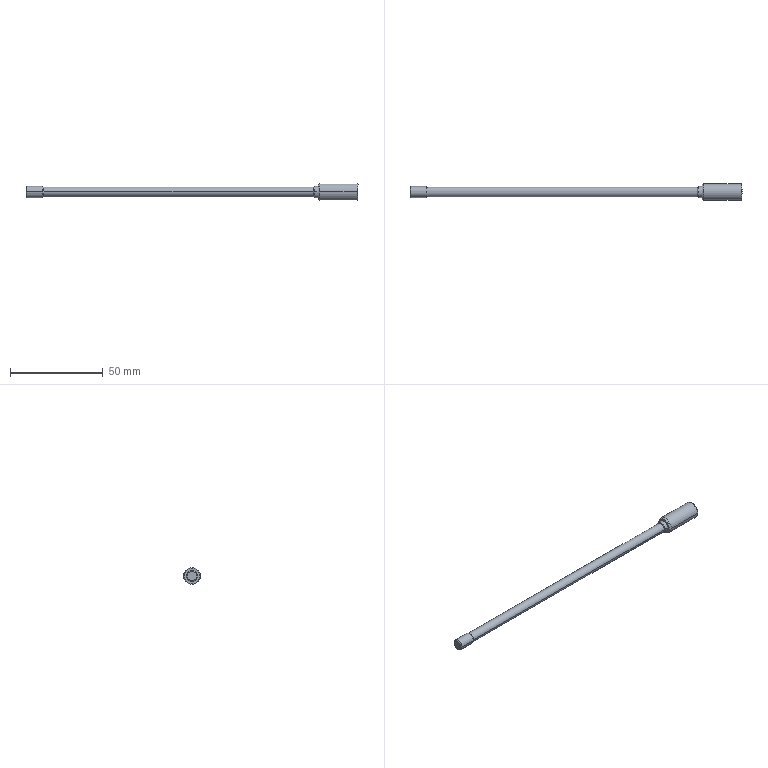Component | SolidWorks | HZ022-SC32x100S-1_HZ022-SC32x100S (5)-1 | 1 solid | 38 faces | box 178.5 x 9 x 9 mm | volume 4474 mm3 | plane 16 | cylinder 10 | cone 10 | spline 2 | commonest cylinder face diameters 6 x4 5.22 x2 9 x2 4.917 x2 | material AL6061
STEP:
#1=COLOUR_RGB('',0.7922,0.8196,0.9333);
#2=FILL_AREA_STYLE_COLOUR('',#1);
#3=FILL_AREA_STYLE('',(#2));
#4=SURFACE_STYLE_FILL_AREA(#3);
#5=SURFACE_SIDE_STYLE('',(#4));
#6=SURFACE_STYLE_USAGE(.BOTH.,#5);
#7=PRESENTATION_STYLE_ASSIGNMENT((#6));
#8=CARTESIAN_POINT('',(-3.546,5.478,37.146));
#9=VERTEX_POINT('',#8);
#10=CARTESIAN_POINT('',(-3.546,5.793,37.146));
#11=VERTEX_POINT('',#10);
#12=CARTESIAN_POINT('',(-3.546,5.478,37.146));
#13=CARTESIAN_POINT('',(-3.546,5.478,37.461));
#14=CARTESIAN_POINT('',(-3.546,5.793,37.461));
#15=CARTESIAN_POINT('',(-3.546,5.793,37.146));
#16=(BOUNDED_CURVE()B_SPLINE_CURVE(3,(#12,#13,#14,#15),.UNSPECIFIED.,.F.,.F.)B_SPLINE_CURVE_WITH_KNOTS((4,4),(0.,1.),.UNSPECIFIED.)CURVE()GEOMETRIC_REPRESENTATION_ITEM()RATIONAL_B_SPLINE_CURVE((1.,0.3333,0.3333,1.))REPRESENTATION_ITEM(''));
#17=EDGE_CURVE('',#9,#11,#16,.T.);
#18=ORIENTED_EDGE('',*,*,#17,.T.);
#19=CARTESIAN_POINT('',(-3.565,5.813,37.146));
#20=VERTEX_POINT('',#19);
#21=CARTESIAN_POINT('',(-3.565,5.793,37.146));
#22=DIRECTION('',(0.,0.,1.));
#23=DIRECTION('',(0.,1.,0.));
#24=AXIS2_PLACEMENT_3D('',#21,#22,#23);
#25=CIRCLE('',#24,0.01969);
#26=EDGE_CURVE('',#11,#20,#25,.T.);
#27=ORIENTED_EDGE('',*,*,#26,.T.);
#28=CARTESIAN_POINT('',(-3.565,5.459,37.146));
#29=VERTEX_POINT('',#28);
#30=CARTESIAN_POINT('',(-3.565,5.636,37.146));
#31=DIRECTION('',(-1.,-0.,0.));
#32=DIRECTION('',(0.,1.,0.));
#33=AXIS2_PLACEMENT_3D('',#30,#31,#32);
#34=CIRCLE('',#33,0.1772);
#35=EDGE_CURVE('',#29,#20,#34,.T.);
#36=ORIENTED_EDGE('',*,*,#35,.F.);
#37=CARTESIAN_POINT('',(-3.565,5.478,37.146));
#38=DIRECTION('',(-0.,0.,-1.));
#39=DIRECTION('',(0.,-1.,0.));
#40=AXIS2_PLACEMENT_3D('',#37,#38,#39);
#41=CIRCLE('',#40,0.01969);
#42=EDGE_CURVE('',#9,#29,#41,.T.);
#43=ORIENTED_EDGE('',*,*,#42,.F.);
#44=EDGE_LOOP('',(#18,#27,#36,#43));
#45=FACE_OUTER_BOUND('',#44,.T.);
#46=CARTESIAN_POINT('',(-3.546,5.793,37.146));
#47=CARTESIAN_POINT('',(-3.546,5.793,37.461));
#48=CARTESIAN_POINT('',(-3.546,5.478,37.461));
#49=CARTESIAN_POINT('',(-3.546,5.478,37.146));
#50=CARTESIAN_POINT('',(-3.546,5.805,37.146));
#51=CARTESIAN_POINT('',(-3.546,5.805,37.484));
#52=CARTESIAN_POINT('',(-3.546,5.467,37.484));
#53=CARTESIAN_POINT('',(-3.546,5.467,37.146));
#54=CARTESIAN_POINT('',(-3.554,5.813,37.146));
#55=CARTESIAN_POINT('',(-3.554,5.813,37.5));
#56=CARTESIAN_POINT('',(-3.554,5.459,37.5));
#57=CARTESIAN_POINT('',(-3.554,5.459,37.146));
#58=CARTESIAN_POINT('',(-3.565,5.813,37.146));
#59=CARTESIAN_POINT('',(-3.565,5.813,37.5));
#60=CARTESIAN_POINT('',(-3.565,5.459,37.5));
#61=CARTESIAN_POINT('',(-3.565,5.459,37.146));
#62=(BOUNDED_SURFACE()B_SPLINE_SURFACE(3,3,((#46,#47,#48,#49),(#50,#51,#52,#53),(#54,#55,#56,#57),(#58,#59,#60,#61)),.UNSPECIFIED.,.F.,.F.,.T.)B_SPLINE_SURFACE_WITH_KNOTS((4,4),(4,4),(0.,1.),(0.,1.),.UNSPECIFIED.)GEOMETRIC_REPRESENTATION_ITEM()RATIONAL_B_SPLINE_SURFACE(((1.,0.3333,0.3333,1.),(0.8047,0.2682,0.2682,0.8047),(0.8047,0.2682,0.2682,0.8047),(1.,0.3333,0.3333,1.)))REPRESENTATION_ITEM('')SURFACE());
#63=ADVANCED_FACE('',(#45),#62,.T.);
#64=CARTESIAN_POINT('',(-4.49,5.739,37.146));
#65=VERTEX_POINT('',#64);
#66=CARTESIAN_POINT('',(-4.49,5.533,37.146));
#67=VERTEX_POINT('',#66);
#68=CARTESIAN_POINT('',(-4.49,5.636,37.146));
#69=DIRECTION('',(-1.,-0.,0.));
#70=DIRECTION('',(0.,1.,0.));
#71=AXIS2_PLACEMENT_3D('',#68,#69,#70);
#72=CIRCLE('',#71,0.1028);
#73=EDGE_CURVE('',#65,#67,#72,.T.);
#74=ORIENTED_EDGE('',*,*,#73,.T.);
#75=CARTESIAN_POINT('',(-10.199,5.533,37.146));
#76=VERTEX_POINT('',#75);
#77=CARTESIAN_POINT('',(-7.345,5.533,37.146));
#78=DIRECTION('',(-1.,-0.,0.));
#79=VECTOR('',#78,39.37);
#80=LINE('',#77,#79);
#81=EDGE_CURVE('',#67,#76,#80,.T.);
#82=ORIENTED_EDGE('',*,*,#81,.T.);
#83=CARTESIAN_POINT('',(-10.199,5.739,37.146));
#84=VERTEX_POINT('',#83);
#85=CARTESIAN_POINT('',(-10.199,5.636,37.146));
#86=DIRECTION('',(1.,0.,-0.));
#87=DIRECTION('',(0.,1.,0.));
#88=AXIS2_PLACEMENT_3D('',#85,#86,#87);
#89=CIRCLE('',#88,0.1028);
#90=EDGE_CURVE('',#76,#84,#89,.T.);
#91=ORIENTED_EDGE('',*,*,#90,.T.);
#92=CARTESIAN_POINT('',(-7.345,5.739,37.146));
#93=DIRECTION('',(-1.,-0.,0.));
#94=VECTOR('',#93,39.37);
#95=LINE('',#92,#94);
#96=EDGE_CURVE('',#65,#84,#95,.T.);
#97=ORIENTED_EDGE('',*,*,#96,.F.);
#98=EDGE_LOOP('',(#74,#82,#91,#97));
#99=FACE_OUTER_BOUND('',#98,.T.);
#100=CARTESIAN_POINT('',(-7.345,5.636,37.146));
#101=DIRECTION('',(-1.,-0.,0.));
#102=DIRECTION('',(0.,1.,0.));
#103=AXIS2_PLACEMENT_3D('',#100,#101,#102);
#104=CYLINDRICAL_SURFACE('',#103,0.1028);
#105=ADVANCED_FACE('',(#99),#104,.T.);
#106=ORIENTED_EDGE('',*,*,#90,.F.);
#107=CARTESIAN_POINT('',(-10.214,5.518,37.146));
#108=VERTEX_POINT('',#107);
#109=CARTESIAN_POINT('',(-10.214,5.518,37.146));
#110=DIRECTION('',(-0.7071,-0.7071,0.));
#111=VECTOR('',#110,39.37);
#112=LINE('',#109,#111);
#113=EDGE_CURVE('',#76,#108,#112,.T.);
#114=ORIENTED_EDGE('',*,*,#113,.T.);
#115=CARTESIAN_POINT('',(-10.214,5.754,37.146));
#116=VERTEX_POINT('',#115);
#117=CARTESIAN_POINT('',(-10.214,5.636,37.146));
#118=DIRECTION('',(1.,0.,-0.));
#119=DIRECTION('',(-0.,0.,-1.));
#120=AXIS2_PLACEMENT_3D('',#117,#118,#119);
#121=CIRCLE('',#120,0.1181);
#122=EDGE_CURVE('',#108,#116,#121,.T.);
#123=ORIENTED_EDGE('',*,*,#122,.T.);
#124=CARTESIAN_POINT('',(-10.214,5.754,37.146));
#125=DIRECTION('',(-0.7071,0.7071,0.));
#126=VECTOR('',#125,39.37);
#127=LINE('',#124,#126);
#128=EDGE_CURVE('',#84,#116,#127,.T.);
#129=ORIENTED_EDGE('',*,*,#128,.F.);
#130=EDGE_LOOP('',(#106,#114,#123,#129));
#131=FACE_OUTER_BOUND('',#130,.T.);
#132=CARTESIAN_POINT('',(-10.214,5.636,37.146));
#133=DIRECTION('',(-1.,-0.,0.));
#134=DIRECTION('',(0.,1.,0.));
#135=AXIS2_PLACEMENT_3D('',#132,#133,#134);
#136=CONICAL_SURFACE('',#135,0.1181,0.7854);
#137=ADVANCED_FACE('',(#131),#136,.T.);
#138=ORIENTED_EDGE('',*,*,#73,.F.);
#139=CARTESIAN_POINT('',(-4.475,5.754,37.146));
#140=VERTEX_POINT('',#139);
#141=CARTESIAN_POINT('',(-4.475,5.754,37.146));
#142=DIRECTION('',(0.7071,0.7071,-0.));
#143=VECTOR('',#142,39.37);
#144=LINE('',#141,#143);
#145=EDGE_CURVE('',#65,#140,#144,.T.);
#146=ORIENTED_EDGE('',*,*,#145,.T.);
#147=CARTESIAN_POINT('',(-4.475,5.518,37.146));
#148=VERTEX_POINT('',#147);
#149=CARTESIAN_POINT('',(-4.475,5.636,37.146));
#150=DIRECTION('',(-1.,-0.,0.));
#151=DIRECTION('',(-0.,0.,-1.));
#152=AXIS2_PLACEMENT_3D('',#149,#150,#151);
#153=CIRCLE('',#152,0.1181);
#154=EDGE_CURVE('',#140,#148,#153,.T.);
#155=ORIENTED_EDGE('',*,*,#154,.T.);
#156=CARTESIAN_POINT('',(-4.475,5.518,37.146));
#157=DIRECTION('',(0.7071,-0.7071,-0.));
#158=VECTOR('',#157,39.37);
#159=LINE('',#156,#158);
#160=EDGE_CURVE('',#67,#148,#159,.T.);
#161=ORIENTED_EDGE('',*,*,#160,.F.);
#162=EDGE_LOOP('',(#138,#146,#155,#161));
#163=FACE_OUTER_BOUND('',#162,.T.);
#164=CARTESIAN_POINT('',(-4.475,5.636,37.146));
#165=DIRECTION('',(1.,-0.,-0.));
#166=DIRECTION('',(0.,-1.,0.));
#167=AXIS2_PLACEMENT_3D('',#164,#165,#166);
#168=CONICAL_SURFACE('',#167,0.1181,0.7854);
#169=ADVANCED_FACE('',(#163),#168,.T.);
#170=ORIENTED_EDGE('',*,*,#122,.F.);
#171=CARTESIAN_POINT('',(-10.553,5.518,37.146));
#172=VERTEX_POINT('',#171);
#173=CARTESIAN_POINT('',(-10.384,5.518,37.146));
#174=DIRECTION('',(-1.,-0.,0.));
#175=VECTOR('',#174,39.37);
#176=LINE('',#173,#175);
#177=EDGE_CURVE('',#108,#172,#176,.T.);
#178=ORIENTED_EDGE('',*,*,#177,.T.);
#179=CARTESIAN_POINT('',(-10.553,5.754,37.146));
#180=VERTEX_POINT('',#179);
#181=CARTESIAN_POINT('',(-10.553,5.636,37.146));
#182=DIRECTION('',(1.,0.,-0.));
#183=DIRECTION('',(0.,1.,0.));
#184=AXIS2_PLACEMENT_3D('',#181,#182,#183);
#185=CIRCLE('',#184,0.1181);
#186=EDGE_CURVE('',#172,#180,#185,.T.);
#187=ORIENTED_EDGE('',*,*,#186,.T.);
#188=CARTESIAN_POINT('',(-10.384,5.754,37.146));
#189=DIRECTION('',(-1.,-0.,0.));
#190=VECTOR('',#189,39.37);
#191=LINE('',#188,#190);
#192=EDGE_CURVE('',#116,#180,#191,.T.);
#193=ORIENTED_EDGE('',*,*,#192,.F.);
#194=EDGE_LOOP('',(#170,#178,#187,#193));
#195=FACE_OUTER_BOUND('',#194,.T.);
#196=CARTESIAN_POINT('',(-10.384,5.636,37.146));
#197=DIRECTION('',(-1.,-0.,0.));
#198=DIRECTION('',(0.,1.,0.));
#199=AXIS2_PLACEMENT_3D('',#196,#197,#198);
#200=CYLINDRICAL_SURFACE('',#199,0.1181);
#201=ADVANCED_FACE('',(#195),#200,.T.);
#202=CARTESIAN_POINT('',(-4.392,5.754,37.146));
#203=VERTEX_POINT('',#202);
#204=CARTESIAN_POINT('',(-4.392,5.518,37.146));
#205=VERTEX_POINT('',#204);
#206=CARTESIAN_POINT('',(-4.392,5.636,37.146));
#207=DIRECTION('',(-1.,-0.,0.));
#208=DIRECTION('',(0.,1.,0.));
#209=AXIS2_PLACEMENT_3D('',#206,#207,#208);
#210=CIRCLE('',#209,0.1181);
#211=EDGE_CURVE('',#203,#205,#210,.T.);
#212=ORIENTED_EDGE('',*,*,#211,.T.);
#213=CARTESIAN_POINT('',(-4.306,5.518,37.146));
#214=DIRECTION('',(-1.,-0.,0.));
#215=VECTOR('',#214,39.37);
#216=LINE('',#213,#215);
#217=EDGE_CURVE('',#205,#148,#216,.T.);
#218=ORIENTED_EDGE('',*,*,#217,.T.);
#219=ORIENTED_EDGE('',*,*,#154,.F.);
#220=CARTESIAN_POINT('',(-4.306,5.754,37.146));
#221=DIRECTION('',(-1.,-0.,0.));
#222=VECTOR('',#221,39.37);
#223=LINE('',#220,#222);
#224=EDGE_CURVE('',#203,#140,#223,.T.);
#225=ORIENTED_EDGE('',*,*,#224,.F.);
#226=EDGE_LOOP('',(#212,#218,#219,#225));
#227=FACE_OUTER_BOUND('',#226,.T.);
#228=CARTESIAN_POINT('',(-4.306,5.636,37.146));
#229=DIRECTION('',(-1.,-0.,0.));
#230=DIRECTION('',(0.,1.,0.));
#231=AXIS2_PLACEMENT_3D('',#228,#229,#230);
#232=CYLINDRICAL_SURFACE('',#231,0.1181);
#233=ADVANCED_FACE('',(#227),#232,.T.);
#234=CARTESIAN_POINT('',(-10.573,5.537,37.146));
#235=VERTEX_POINT('',#234);
#236=CARTESIAN_POINT('',(-10.573,5.734,37.146));
#237=VERTEX_POINT('',#236);
#238=CARTESIAN_POINT('',(-10.573,5.636,37.146));
#239=DIRECTION('',(1.,0.,-0.));
#240=DIRECTION('',(0.,-1.,0.));
#241=AXIS2_PLACEMENT_3D('',#238,#239,#240);
#242=CIRCLE('',#241,0.09843);
#243=EDGE_CURVE('',#235,#237,#242,.T.);
#244=ORIENTED_EDGE('',*,*,#243,.T.);
#245=CARTESIAN_POINT('',(-10.553,5.754,37.146));
#246=DIRECTION('',(0.7071,0.7071,-0.));
#247=VECTOR('',#246,39.37);
#248=LINE('',#245,#247);
#249=EDGE_CURVE('',#237,#180,#248,.T.);
#250=ORIENTED_EDGE('',*,*,#249,.T.);
#251=ORIENTED_EDGE('',*,*,#186,.F.);
#252=CARTESIAN_POINT('',(-10.553,5.518,37.146));
#253=DIRECTION('',(0.7071,-0.7071,-0.));
#254=VECTOR('',#253,39.37);
#255=LINE('',#252,#254);
#256=EDGE_CURVE('',#235,#172,#255,.T.);
#257=ORIENTED_EDGE('',*,*,#256,.F.);
#258=EDGE_LOOP('',(#244,#250,#251,#257));
#259=FACE_OUTER_BOUND('',#258,.T.);
#260=CARTESIAN_POINT('',(-10.553,5.636,37.146));
#261=DIRECTION('',(1.,0.,-0.));
#262=DIRECTION('',(0.,-1.,0.));
#263=AXIS2_PLACEMENT_3D('',#260,#261,#262);
#264=CONICAL_SURFACE('',#263,0.1181,0.7854);
#265=ADVANCED_FACE('',(#259),#264,.T.);
#266=CARTESIAN_POINT('',(-4.392,5.803,37.146));
#267=VERTEX_POINT('',#266);
#268=CARTESIAN_POINT('',(-4.392,5.469,37.146));
#269=VERTEX_POINT('',#268);
#270=CARTESIAN_POINT('',(-4.392,5.636,37.146));
#271=DIRECTION('',(-1.,-0.,0.));
#272=DIRECTION('',(0.,-1.,0.));
#273=AXIS2_PLACEMENT_3D('',#270,#271,#272);
#274=CIRCLE('',#273,0.1666);
#275=EDGE_CURVE('',#267,#269,#274,.T.);
#276=ORIENTED_EDGE('',*,*,#275,.F.);
#277=CARTESIAN_POINT('',(-4.353,5.813,37.146));
#278=VERTEX_POINT('',#277);
#279=CARTESIAN_POINT('',(-4.353,5.813,37.146));
#280=DIRECTION('',(0.9659,0.2588,-0.));
#281=VECTOR('',#280,39.37);
#282=LINE('',#279,#281);
#283=EDGE_CURVE('',#267,#278,#282,.T.);
#284=ORIENTED_EDGE('',*,*,#283,.T.);
#285=CARTESIAN_POINT('',(-4.353,5.459,37.146));
#286=VERTEX_POINT('',#285);
#287=CARTESIAN_POINT('',(-4.353,5.636,37.146));
#288=DIRECTION('',(-1.,-0.,0.));
#289=DIRECTION('',(-0.,0.,-1.));
#290=AXIS2_PLACEMENT_3D('',#287,#288,#289);
#291=CIRCLE('',#290,0.1772);
#292=EDGE_CURVE('',#278,#286,#291,.T.);
#293=ORIENTED_EDGE('',*,*,#292,.T.);
#294=CARTESIAN_POINT('',(-4.353,5.459,37.146));
#295=DIRECTION('',(0.9659,-0.2588,-0.));
#296=VECTOR('',#295,39.37);
#297=LINE('',#294,#296);
#298=EDGE_CURVE('',#269,#286,#297,.T.);
#299=ORIENTED_EDGE('',*,*,#298,.F.);
#300=EDGE_LOOP('',(#276,#284,#293,#299));
#301=FACE_OUTER_BOUND('',#300,.T.);
#302=CARTESIAN_POINT('',(-4.353,5.636,37.146));
#303=DIRECTION('',(1.,0.,-0.));
#304=DIRECTION('',(0.,-1.,0.));
#305=AXIS2_PLACEMENT_3D('',#302,#303,#304);
#306=CONICAL_SURFACE('',#305,0.1772,0.2618);
#307=ADVANCED_FACE('',(#301),#306,.T.);
#308=CARTESIAN_POINT('',(-3.565,5.636,37.146));
#309=DIRECTION('',(-1.,-0.,0.));
#310=DIRECTION('',(0.,1.,0.));
#311=AXIS2_PLACEMENT_3D('',#308,#309,#310);
#312=CIRCLE('',#311,0.1772);
#313=EDGE_CURVE('',#20,#29,#312,.T.);
#314=ORIENTED_EDGE('',*,*,#313,.T.);
#315=CARTESIAN_POINT('',(-3.959,5.459,37.146));
#316=DIRECTION('',(-1.,-0.,0.));
#317=VECTOR('',#316,39.37);
#318=LINE('',#315,#317);
#319=EDGE_CURVE('',#29,#286,#318,.T.);
#320=ORIENTED_EDGE('',*,*,#319,.T.);
#321=ORIENTED_EDGE('',*,*,#292,.F.);
#322=CARTESIAN_POINT('',(-3.959,5.813,37.146));
#323=DIRECTION('',(-1.,-0.,0.));
#324=VECTOR('',#323,39.37);
#325=LINE('',#322,#324);
#326=EDGE_CURVE('',#20,#278,#325,.T.);
#327=ORIENTED_EDGE('',*,*,#326,.F.);
#328=EDGE_LOOP('',(#314,#320,#321,#327));
#329=FACE_OUTER_BOUND('',#328,.T.);
#330=CARTESIAN_POINT('',(-3.959,5.636,37.146));
#331=DIRECTION('',(-1.,-0.,0.));
#332=DIRECTION('',(0.,1.,0.));
#333=AXIS2_PLACEMENT_3D('',#330,#331,#332);
#334=CYLINDRICAL_SURFACE('',#333,0.1772);
#335=ADVANCED_FACE('',(#329),#334,.T.);
#336=CARTESIAN_POINT('',(-3.724,5.733,37.146));
#337=VERTEX_POINT('',#336);
#338=CARTESIAN_POINT('',(-3.724,5.539,37.146));
#339=VERTEX_POINT('',#338);
#340=CARTESIAN_POINT('',(-3.724,5.636,37.146));
#341=DIRECTION('',(1.,0.,-0.));
#342=DIRECTION('',(-0.,0.,-1.));
#343=AXIS2_PLACEMENT_3D('',#340,#341,#342);
#344=CIRCLE('',#343,0.09679);
#345=EDGE_CURVE('',#337,#339,#344,.T.);
#346=ORIENTED_EDGE('',*,*,#345,.F.);
#347=CARTESIAN_POINT('',(-3.703,5.754,37.146));
#348=VERTEX_POINT('',#347);
#349=CARTESIAN_POINT('',(-3.703,5.754,37.146));
#350=DIRECTION('',(0.7071,0.7071,-0.));
#351=VECTOR('',#350,39.37);
#352=LINE('',#349,#351);
#353=EDGE_CURVE('',#337,#348,#352,.T.);
#354=ORIENTED_EDGE('',*,*,#353,.T.);
#355=CARTESIAN_POINT('',(-3.703,5.695,37.248));
#356=VERTEX_POINT('',#355);
#357=CARTESIAN_POINT('',(-3.703,5.636,37.146));
#358=DIRECTION('',(-1.,-0.,0.));
#359=DIRECTION('',(0.,-1.,0.));
#360=AXIS2_PLACEMENT_3D('',#357,#358,#359);
#361=CIRCLE('',#360,0.1181);
#362=EDGE_CURVE('',#356,#348,#361,.T.);
#363=ORIENTED_EDGE('',*,*,#362,.F.);
#364=CARTESIAN_POINT('',(-3.703,5.577,37.248));
#365=VERTEX_POINT('',#364);
#366=CARTESIAN_POINT('',(-3.703,5.636,37.146));
#367=DIRECTION('',(-1.,-0.,0.));
#368=DIRECTION('',(0.,-1.,0.));
#369=AXIS2_PLACEMENT_3D('',#366,#367,#368);
#370=CIRCLE('',#369,0.1181);
#371=EDGE_CURVE('',#365,#356,#370,.T.);
#372=ORIENTED_EDGE('',*,*,#371,.F.);
#373=CARTESIAN_POINT('',(-3.703,5.518,37.146));
#374=VERTEX_POINT('',#373);
#375=CARTESIAN_POINT('',(-3.703,5.636,37.146));
#376=DIRECTION('',(-1.,-0.,0.));
#377=DIRECTION('',(0.,-1.,0.));
#378=AXIS2_PLACEMENT_3D('',#375,#376,#377);
#379=CIRCLE('',#378,0.1181);
#380=EDGE_CURVE('',#374,#365,#379,.T.);
#381=ORIENTED_EDGE('',*,*,#380,.F.);
#382=CARTESIAN_POINT('',(-3.703,5.518,37.146));
#383=DIRECTION('',(0.7071,-0.7071,-0.));
#384=VECTOR('',#383,39.37);
#385=LINE('',#382,#384);
#386=EDGE_CURVE('',#339,#374,#385,.T.);
#387=ORIENTED_EDGE('',*,*,#386,.F.);
#388=EDGE_LOOP('',(#346,#354,#363,#372,#381,#387));
#389=FACE_OUTER_BOUND('',#388,.T.);
#390=CARTESIAN_POINT('',(-3.703,5.636,37.146));
#391=DIRECTION('',(1.,0.,-0.));
#392=DIRECTION('',(0.,-1.,0.));
#393=AXIS2_PLACEMENT_3D('',#390,#391,#392);
#394=CONICAL_SURFACE('',#393,0.1181,0.7854);
#395=ADVANCED_FACE('',(#389),#394,.F.);
#396=ORIENTED_EDGE('',*,*,#345,.T.);
#397=CARTESIAN_POINT('',(-4.116,5.539,37.146));
#398=VERTEX_POINT('',#397);
#399=CARTESIAN_POINT('',(-4.047,5.539,37.146));
#400=DIRECTION('',(-1.,-0.,0.));
#401=VECTOR('',#400,39.37);
#402=LINE('',#399,#401);
#403=EDGE_CURVE('',#339,#398,#402,.T.);
#404=ORIENTED_EDGE('',*,*,#403,.T.);
#405=CARTESIAN_POINT('',(-4.116,5.733,37.146));
#406=VERTEX_POINT('',#405);
#407=CARTESIAN_POINT('',(-4.116,5.636,37.146));
#408=DIRECTION('',(1.,0.,-0.));
#409=DIRECTION('',(0.,1.,0.));
#410=AXIS2_PLACEMENT_3D('',#407,#408,#409);
#411=CIRCLE('',#410,0.09679);
#412=EDGE_CURVE('',#406,#398,#411,.T.);
#413=ORIENTED_EDGE('',*,*,#412,.F.);
#414=CARTESIAN_POINT('',(-4.047,5.733,37.146));
#415=DIRECTION('',(-1.,-0.,0.));
#416=VECTOR('',#415,39.37);
#417=LINE('',#414,#416);
#418=EDGE_CURVE('',#337,#406,#417,.T.);
#419=ORIENTED_EDGE('',*,*,#418,.F.);
#420=EDGE_LOOP('',(#396,#404,#413,#419));
#421=FACE_OUTER_BOUND('',#420,.T.);
#422=CARTESIAN_POINT('',(-4.047,5.636,37.146));
#423=DIRECTION('',(-1.,-0.,0.));
#424=DIRECTION('',(0.,1.,0.));
#425=AXIS2_PLACEMENT_3D('',#422,#423,#424);
#426=CYLINDRICAL_SURFACE('',#425,0.09679);
#427=ADVANCED_FACE('',(#421),#426,.F.);
#428=ORIENTED_EDGE('',*,*,#81,.F.);
#429=CARTESIAN_POINT('',(-4.49,5.636,37.146));
#430=DIRECTION('',(-1.,-0.,0.));
#431=DIRECTION('',(0.,1.,0.));
#432=AXIS2_PLACEMENT_3D('',#429,#430,#431);
#433=CIRCLE('',#432,0.1028);
#434=EDGE_CURVE('',#67,#65,#433,.T.);
#435=ORIENTED_EDGE('',*,*,#434,.T.);
#436=ORIENTED_EDGE('',*,*,#96,.T.);
#437=CARTESIAN_POINT('',(-10.199,5.636,37.146));
#438=DIRECTION('',(1.,0.,-0.));
#439=DIRECTION('',(0.,1.,0.));
#440=AXIS2_PLACEMENT_3D('',#437,#438,#439);
#441=CIRCLE('',#440,0.1028);
#442=EDGE_CURVE('',#84,#76,#441,.T.);
#443=ORIENTED_EDGE('',*,*,#442,.T.);
#444=EDGE_LOOP('',(#428,#435,#436,#443));
#445=FACE_OUTER_BOUND('',#444,.T.);
#446=CARTESIAN_POINT('',(-7.345,5.636,37.146));
#447=DIRECTION('',(-1.,-0.,0.));
#448=DIRECTION('',(0.,1.,0.));
#449=AXIS2_PLACEMENT_3D('',#446,#447,#448);
#450=CYLINDRICAL_SURFACE('',#449,0.1028);
#451=ADVANCED_FACE('',(#445),#450,.T.);
#452=ORIENTED_EDGE('',*,*,#113,.F.);
#453=ORIENTED_EDGE('',*,*,#442,.F.);
#454=ORIENTED_EDGE('',*,*,#128,.T.);
#455=CARTESIAN_POINT('',(-10.214,5.636,37.146));
#456=DIRECTION('',(1.,0.,-0.));
#457=DIRECTION('',(-0.,0.,-1.));
#458=AXIS2_PLACEMENT_3D('',#455,#456,#457);
#459=CIRCLE('',#458,0.1181);
#460=EDGE_CURVE('',#116,#108,#459,.T.);
#461=ORIENTED_EDGE('',*,*,#460,.T.);
#462=EDGE_LOOP('',(#452,#453,#454,#461));
#463=FACE_OUTER_BOUND('',#462,.T.);
#464=CARTESIAN_POINT('',(-10.214,5.636,37.146));
#465=DIRECTION('',(-1.,-0.,0.));
#466=DIRECTION('',(0.,1.,0.));
#467=AXIS2_PLACEMENT_3D('',#464,#465,#466);
#468=CONICAL_SURFACE('',#467,0.1181,0.7854);
#469=ADVANCED_FACE('',(#463),#468,.T.);
#470=ORIENTED_EDGE('',*,*,#145,.F.);
#471=ORIENTED_EDGE('',*,*,#434,.F.);
#472=ORIENTED_EDGE('',*,*,#160,.T.);
#473=CARTESIAN_POINT('',(-4.475,5.636,37.146));
#474=DIRECTION('',(-1.,-0.,0.));
#475=DIRECTION('',(-0.,0.,-1.));
#476=AXIS2_PLACEMENT_3D('',#473,#474,#475);
#477=CIRCLE('',#476,0.1181);
#478=EDGE_CURVE('',#148,#140,#477,.T.);
#479=ORIENTED_EDGE('',*,*,#478,.T.);
#480=EDGE_LOOP('',(#470,#471,#472,#479));
#481=FACE_OUTER_BOUND('',#480,.T.);
#482=CARTESIAN_POINT('',(-4.475,5.636,37.146));
#483=DIRECTION('',(1.,-0.,-0.));
#484=DIRECTION('',(0.,-1.,0.));
#485=AXIS2_PLACEMENT_3D('',#482,#483,#484);
#486=CONICAL_SURFACE('',#485,0.1181,0.7854);
#487=ADVANCED_FACE('',(#481),#486,.T.);
#488=ORIENTED_EDGE('',*,*,#177,.F.);
#489=ORIENTED_EDGE('',*,*,#460,.F.);
#490=ORIENTED_EDGE('',*,*,#192,.T.);
#491=CARTESIAN_POINT('',(-10.553,5.636,37.146));
#492=DIRECTION('',(1.,0.,-0.));
#493=DIRECTION('',(0.,1.,0.));
#494=AXIS2_PLACEMENT_3D('',#491,#492,#493);
#495=CIRCLE('',#494,0.1181);
#496=EDGE_CURVE('',#180,#172,#495,.T.);
#497=ORIENTED_EDGE('',*,*,#496,.T.);
#498=EDGE_LOOP('',(#488,#489,#490,#497));
#499=FACE_OUTER_BOUND('',#498,.T.);
#500=CARTESIAN_POINT('',(-10.384,5.636,37.146));
#501=DIRECTION('',(-1.,-0.,0.));
#502=DIRECTION('',(0.,1.,0.));
#503=AXIS2_PLACEMENT_3D('',#500,#501,#502);
#504=CYLINDRICAL_SURFACE('',#503,0.1181);
#505=ADVANCED_FACE('',(#499),#504,.T.);
#506=ORIENTED_EDGE('',*,*,#217,.F.);
#507=CARTESIAN_POINT('',(-4.392,5.636,37.146));
#508=DIRECTION('',(-1.,-0.,0.));
#509=DIRECTION('',(0.,1.,0.));
#510=AXIS2_PLACEMENT_3D('',#507,#508,#509);
#511=CIRCLE('',#510,0.1181);
#512=EDGE_CURVE('',#205,#203,#511,.T.);
#513=ORIENTED_EDGE('',*,*,#512,.T.);
#514=ORIENTED_EDGE('',*,*,#224,.T.);
#515=ORIENTED_EDGE('',*,*,#478,.F.);
#516=EDGE_LOOP('',(#506,#513,#514,#515));
#517=FACE_OUTER_BOUND('',#516,.T.);
#518=CARTESIAN_POINT('',(-4.306,5.636,37.146));
#519=DIRECTION('',(-1.,-0.,0.));
#520=DIRECTION('',(0.,1.,0.));
#521=AXIS2_PLACEMENT_3D('',#518,#519,#520);
#522=CYLINDRICAL_SURFACE('',#521,0.1181);
#523=ADVANCED_FACE('',(#517),#522,.T.);
#524=ORIENTED_EDGE('',*,*,#249,.F.);
#525=CARTESIAN_POINT('',(-10.573,5.636,37.146));
#526=DIRECTION('',(1.,0.,-0.));
#527=DIRECTION('',(0.,-1.,0.));
#528=AXIS2_PLACEMENT_3D('',#525,#526,#527);
#529=CIRCLE('',#528,0.09843);
#530=EDGE_CURVE('',#237,#235,#529,.T.);
#531=ORIENTED_EDGE('',*,*,#530,.T.);
#532=ORIENTED_EDGE('',*,*,#256,.T.);
#533=ORIENTED_EDGE('',*,*,#496,.F.);
#534=EDGE_LOOP('',(#524,#531,#532,#533));
#535=FACE_OUTER_BOUND('',#534,.T.);
#536=CARTESIAN_POINT('',(-10.553,5.636,37.146));
#537=DIRECTION('',(1.,0.,-0.));
#538=DIRECTION('',(0.,-1.,0.));
#539=AXIS2_PLACEMENT_3D('',#536,#537,#538);
#540=CONICAL_SURFACE('',#539,0.1181,0.7854);
#541=ADVANCED_FACE('',(#535),#540,.T.);
#542=CARTESIAN_POINT('',(-4.392,5.636,37.146));
#543=DIRECTION('',(-1.,-0.,0.));
#544=DIRECTION('',(0.,-1.,0.));
#545=AXIS2_PLACEMENT_3D('',#542,#543,#544);
#546=CIRCLE('',#545,0.1666);
#547=EDGE_CURVE('',#269,#267,#546,.T.);
#548=ORIENTED_EDGE('',*,*,#547,.T.);
#549=ORIENTED_EDGE('',*,*,#275,.T.);
#550=EDGE_LOOP('',(#548,#549));
#551=FACE_OUTER_BOUND('',#550,.T.);
#552=ORIENTED_EDGE('',*,*,#211,.F.);
#553=ORIENTED_EDGE('',*,*,#512,.F.);
#554=EDGE_LOOP('',(#552,#553));
#555=FACE_BOUND('',#554,.T.);
#556=CARTESIAN_POINT('',(-4.392,5.636,37.062));
#557=DIRECTION('',(-1.,-0.,0.));
#558=DIRECTION('',(-0.,1.,0.));
#559=AXIS2_PLACEMENT_3D('',#556,#557,#558);
#560=PLANE('',#559);
#561=ADVANCED_FACE('',(#551,#555),#560,.T.);
#562=ORIENTED_EDGE('',*,*,#243,.F.);
#563=ORIENTED_EDGE('',*,*,#530,.F.);
#564=EDGE_LOOP('',(#562,#563));
#565=FACE_OUTER_BOUND('',#564,.T.);
#566=CARTESIAN_POINT('',(-10.573,5.636,37.096));
#567=DIRECTION('',(-1.,-0.,0.));
#568=DIRECTION('',(-0.,1.,0.));
#569=AXIS2_PLACEMENT_3D('',#566,#567,#568);
#570=PLANE('',#569);
#571=ADVANCED_FACE('',(#565),#570,.T.);
#572=ORIENTED_EDGE('',*,*,#283,.F.);
#573=ORIENTED_EDGE('',*,*,#547,.F.);
#574=ORIENTED_EDGE('',*,*,#298,.T.);
#575=CARTESIAN_POINT('',(-4.353,5.636,37.146));
#576=DIRECTION('',(-1.,-0.,0.));
#577=DIRECTION('',(-0.,0.,-1.));
#578=AXIS2_PLACEMENT_3D('',#575,#576,#577);
#579=CIRCLE('',#578,0.1772);
#580=EDGE_CURVE('',#286,#278,#579,.T.);
#581=ORIENTED_EDGE('',*,*,#580,.T.);
#582=EDGE_LOOP('',(#572,#573,#574,#581));
#583=FACE_OUTER_BOUND('',#582,.T.);
#584=CARTESIAN_POINT('',(-4.353,5.636,37.146));
#585=DIRECTION('',(1.,0.,-0.));
#586=DIRECTION('',(0.,-1.,0.));
#587=AXIS2_PLACEMENT_3D('',#584,#585,#586);
#588=CONICAL_SURFACE('',#587,0.1772,0.2618);
#589=ADVANCED_FACE('',(#583),#588,.T.);
#590=ORIENTED_EDGE('',*,*,#319,.F.);
#591=ORIENTED_EDGE('',*,*,#35,.T.);
#592=ORIENTED_EDGE('',*,*,#326,.T.);
#593=ORIENTED_EDGE('',*,*,#580,.F.);
#594=EDGE_LOOP('',(#590,#591,#592,#593));
#595=FACE_OUTER_BOUND('',#594,.T.);
#596=CARTESIAN_POINT('',(-3.959,5.636,37.146));
#597=DIRECTION('',(-1.,-0.,0.));
#598=DIRECTION('',(0.,1.,0.));
#599=AXIS2_PLACEMENT_3D('',#596,#597,#598);
#600=CYLINDRICAL_SURFACE('',#599,0.1772);
#601=ADVANCED_FACE('',(#595),#600,.T.);
#602=ORIENTED_EDGE('',*,*,#26,.F.);
#603=CARTESIAN_POINT('',(-3.546,5.636,36.988));
#604=VERTEX_POINT('',#603);
#605=CARTESIAN_POINT('',(-3.546,5.793,37.146));
#606=CARTESIAN_POINT('',(-3.546,5.793,37.053));
#607=CARTESIAN_POINT('',(-3.546,5.728,36.988));
#608=CARTESIAN_POINT('',(-3.546,5.636,36.988));
#609=(BOUNDED_CURVE()B_SPLINE_CURVE(3,(#605,#606,#607,#608),.UNSPECIFIED.,.F.,.T.)B_SPLINE_CURVE_WITH_KNOTS((4,4),(0.,1.),.UNSPECIFIED.)CURVE()GEOMETRIC_REPRESENTATION_ITEM()RATIONAL_B_SPLINE_CURVE((1.,0.8047,0.8047,1.))REPRESENTATION_ITEM(''));
#610=EDGE_CURVE('',#11,#604,#609,.T.);
#611=ORIENTED_EDGE('',*,*,#610,.T.);
#612=CARTESIAN_POINT('',(-3.546,5.636,36.988));
#613=CARTESIAN_POINT('',(-3.546,5.544,36.988));
#614=CARTESIAN_POINT('',(-3.546,5.478,37.053));
#615=CARTESIAN_POINT('',(-3.546,5.478,37.146));
#616=(BOUNDED_CURVE()B_SPLINE_CURVE(3,(#612,#613,#614,#615),.UNSPECIFIED.,.F.,.F.)B_SPLINE_CURVE_WITH_KNOTS((4,4),(0.,1.),.UNSPECIFIED.)CURVE()GEOMETRIC_REPRESENTATION_ITEM()RATIONAL_B_SPLINE_CURVE((1.,0.8047,0.8047,1.))REPRESENTATION_ITEM(''));
#617=EDGE_CURVE('',#604,#9,#616,.T.);
#618=ORIENTED_EDGE('',*,*,#617,.T.);
#619=ORIENTED_EDGE('',*,*,#42,.T.);
#620=ORIENTED_EDGE('',*,*,#313,.F.);
#621=EDGE_LOOP('',(#602,#611,#618,#619,#620));
#622=FACE_OUTER_BOUND('',#621,.T.);
#623=CARTESIAN_POINT('',(-3.546,5.478,37.146));
#624=CARTESIAN_POINT('',(-3.546,5.478,36.831));
#625=CARTESIAN_POINT('',(-3.546,5.793,36.831));
#626=CARTESIAN_POINT('',(-3.546,5.793,37.146));
#627=CARTESIAN_POINT('',(-3.546,5.467,37.146));
#628=CARTESIAN_POINT('',(-3.546,5.467,36.808));
#629=CARTESIAN_POINT('',(-3.546,5.805,36.808));
#630=CARTESIAN_POINT('',(-3.546,5.805,37.146));
#631=CARTESIAN_POINT('',(-3.554,5.459,37.146));
#632=CARTESIAN_POINT('',(-3.554,5.459,36.791));
#633=CARTESIAN_POINT('',(-3.554,5.813,36.791));
#634=CARTESIAN_POINT('',(-3.554,5.813,37.146));
#635=CARTESIAN_POINT('',(-3.565,5.459,37.146));
#636=CARTESIAN_POINT('',(-3.565,5.459,36.791));
#637=CARTESIAN_POINT('',(-3.565,5.813,36.791));
#638=CARTESIAN_POINT('',(-3.565,5.813,37.146));
#639=(BOUNDED_SURFACE()B_SPLINE_SURFACE(3,3,((#623,#624,#625,#626),(#627,#628,#629,#630),(#631,#632,#633,#634),(#635,#636,#637,#638)),.UNSPECIFIED.,.F.,.F.,.T.)B_SPLINE_SURFACE_WITH_KNOTS((4,4),(4,4),(0.,1.),(0.,1.),.UNSPECIFIED.)GEOMETRIC_REPRESENTATION_ITEM()RATIONAL_B_SPLINE_SURFACE(((1.,0.3333,0.3333,1.),(0.8047,0.2682,0.2682,0.8047),(0.8047,0.2682,0.2682,0.8047),(1.,0.3333,0.3333,1.)))REPRESENTATION_ITEM('')SURFACE());
#640=ADVANCED_FACE('',(#622),#639,.T.);
#641=ORIENTED_EDGE('',*,*,#17,.F.);
#642=ORIENTED_EDGE('',*,*,#617,.F.);
#643=ORIENTED_EDGE('',*,*,#610,.F.);
#644=EDGE_LOOP('',(#641,#642,#643));
#645=FACE_OUTER_BOUND('',#644,.T.);
#646=CARTESIAN_POINT('',(-3.546,5.754,37.214));
#647=VERTEX_POINT('',#646);
#648=CARTESIAN_POINT('',(-3.546,5.754,37.077));
#649=VERTEX_POINT('',#648);
#650=CARTESIAN_POINT('',(-3.546,5.754,37.067));
#651=DIRECTION('',(-0.,0.,-1.));
#652=VECTOR('',#651,39.37);
#653=LINE('',#650,#652);
#654=EDGE_CURVE('',#647,#649,#653,.T.);
#655=ORIENTED_EDGE('',*,*,#654,.T.);
#656=CARTESIAN_POINT('',(-3.546,5.636,37.009));
#657=VERTEX_POINT('',#656);
#658=CARTESIAN_POINT('',(-3.546,5.754,37.077));
#659=DIRECTION('',(-0.,-0.866,-0.5));
#660=VECTOR('',#659,39.37);
#661=LINE('',#658,#660);
#662=EDGE_CURVE('',#649,#657,#661,.T.);
#663=ORIENTED_EDGE('',*,*,#662,.T.);
#664=CARTESIAN_POINT('',(-3.546,5.518,37.077));
#665=VERTEX_POINT('',#664);
#666=CARTESIAN_POINT('',(-3.546,5.636,37.009));
#667=DIRECTION('',(0.,-0.866,0.5));
#668=VECTOR('',#667,39.37);
#669=LINE('',#666,#668);
#670=EDGE_CURVE('',#657,#665,#669,.T.);
#671=ORIENTED_EDGE('',*,*,#670,.T.);
#672=CARTESIAN_POINT('',(-3.546,5.518,37.214));
#673=VERTEX_POINT('',#672);
#674=CARTESIAN_POINT('',(-3.546,5.518,37.067));
#675=DIRECTION('',(0.,-0.,1.));
#676=VECTOR('',#675,39.37);
#677=LINE('',#674,#676);
#678=EDGE_CURVE('',#665,#673,#677,.T.);
#679=ORIENTED_EDGE('',*,*,#678,.T.);
#680=CARTESIAN_POINT('',(-3.546,5.636,37.282));
#681=VERTEX_POINT('',#680);
#682=CARTESIAN_POINT('',(-3.546,5.518,37.214));
#683=DIRECTION('',(0.,0.866,0.5));
#684=VECTOR('',#683,39.37);
#685=LINE('',#682,#684);
#686=EDGE_CURVE('',#673,#681,#685,.T.);
#687=ORIENTED_EDGE('',*,*,#686,.T.);
#688=CARTESIAN_POINT('',(-3.546,5.636,37.282));
#689=DIRECTION('',(-0.,0.866,-0.5));
#690=VECTOR('',#689,39.37);
#691=LINE('',#688,#690);
#692=EDGE_CURVE('',#681,#647,#691,.T.);
#693=ORIENTED_EDGE('',*,*,#692,.T.);
#694=EDGE_LOOP('',(#655,#663,#671,#679,#687,#693));
#695=FACE_BOUND('',#694,.T.);
#696=CARTESIAN_POINT('',(-3.546,5.636,37.067));
#697=DIRECTION('',(1.,0.,-0.));
#698=DIRECTION('',(0.,-1.,-0.));
#699=AXIS2_PLACEMENT_3D('',#696,#697,#698);
#700=PLANE('',#699);
#701=ADVANCED_FACE('',(#645,#695),#700,.T.);
#702=CARTESIAN_POINT('',(-3.703,5.636,37.009));
#703=VERTEX_POINT('',#702);
#704=CARTESIAN_POINT('',(-3.546,5.636,37.009));
#705=DIRECTION('',(-1.,-0.,0.));
#706=VECTOR('',#705,39.37);
#707=LINE('',#704,#706);
#708=EDGE_CURVE('',#657,#703,#707,.T.);
#709=ORIENTED_EDGE('',*,*,#708,.F.);
#710=ORIENTED_EDGE('',*,*,#662,.F.);
#711=CARTESIAN_POINT('',(-3.703,5.754,37.077));
#712=VERTEX_POINT('',#711);
#713=CARTESIAN_POINT('',(-3.546,5.754,37.077));
#714=DIRECTION('',(1.,0.,-0.));
#715=VECTOR('',#714,39.37);
#716=LINE('',#713,#715);
#717=EDGE_CURVE('',#712,#649,#716,.T.);
#718=ORIENTED_EDGE('',*,*,#717,.F.);
#719=CARTESIAN_POINT('',(-3.703,5.695,37.043));
#720=VERTEX_POINT('',#719);
#721=CARTESIAN_POINT('',(-3.703,5.754,37.077));
#722=DIRECTION('',(-0.,-0.866,-0.5));
#723=VECTOR('',#722,39.37);
#724=LINE('',#721,#723);
#725=EDGE_CURVE('',#712,#720,#724,.T.);
#726=ORIENTED_EDGE('',*,*,#725,.T.);
#727=CARTESIAN_POINT('',(-3.703,5.636,37.009));
#728=DIRECTION('',(0.,0.866,0.5));
#729=VECTOR('',#728,39.37);
#730=LINE('',#727,#729);
#731=EDGE_CURVE('',#703,#720,#730,.T.);
#732=ORIENTED_EDGE('',*,*,#731,.F.);
#733=EDGE_LOOP('',(#709,#710,#718,#726,#732));
#734=FACE_OUTER_BOUND('',#733,.T.);
#735=CARTESIAN_POINT('',(-3.546,5.636,37.009));
#736=DIRECTION('',(-0.,0.5,-0.866));
#737=DIRECTION('',(-0.,-0.866,-0.5));
#738=AXIS2_PLACEMENT_3D('',#735,#736,#737);
#739=PLANE('',#738);
#740=ADVANCED_FACE('',(#734),#739,.F.);
#741=ORIENTED_EDGE('',*,*,#717,.T.);
#742=ORIENTED_EDGE('',*,*,#654,.F.);
#743=CARTESIAN_POINT('',(-3.703,5.754,37.214));
#744=VERTEX_POINT('',#743);
#745=CARTESIAN_POINT('',(-3.546,5.754,37.214));
#746=DIRECTION('',(1.,0.,-0.));
#747=VECTOR('',#746,39.37);
#748=LINE('',#745,#747);
#749=EDGE_CURVE('',#744,#647,#748,.T.);
#750=ORIENTED_EDGE('',*,*,#749,.F.);
#751=CARTESIAN_POINT('',(-3.703,5.754,37.146));
#752=DIRECTION('',(-0.,0.,-1.));
#753=VECTOR('',#752,39.37);
#754=LINE('',#751,#753);
#755=EDGE_CURVE('',#744,#348,#754,.T.);
#756=ORIENTED_EDGE('',*,*,#755,.T.);
#757=CARTESIAN_POINT('',(-3.703,5.754,37.146));
#758=DIRECTION('',(-0.,0.,-1.));
#759=VECTOR('',#758,39.37);
#760=LINE('',#757,#759);
#761=EDGE_CURVE('',#348,#712,#760,.T.);
#762=ORIENTED_EDGE('',*,*,#761,.T.);
#763=EDGE_LOOP('',(#741,#742,#750,#756,#762));
#764=FACE_OUTER_BOUND('',#763,.T.);
#765=CARTESIAN_POINT('',(-3.546,5.754,37.077));
#766=DIRECTION('',(-0.,1.,0.));
#767=DIRECTION('',(1.,0.,-0.));
#768=AXIS2_PLACEMENT_3D('',#765,#766,#767);
#769=PLANE('',#768);
#770=ADVANCED_FACE('',(#764),#769,.F.);
#771=ORIENTED_EDGE('',*,*,#749,.T.);
#772=ORIENTED_EDGE('',*,*,#692,.F.);
#773=CARTESIAN_POINT('',(-3.703,5.636,37.282));
#774=VERTEX_POINT('',#773);
#775=CARTESIAN_POINT('',(-3.546,5.636,37.282));
#776=DIRECTION('',(1.,0.,-0.));
#777=VECTOR('',#776,39.37);
#778=LINE('',#775,#777);
#779=EDGE_CURVE('',#774,#681,#778,.T.);
#780=ORIENTED_EDGE('',*,*,#779,.F.);
#781=CARTESIAN_POINT('',(-3.703,5.754,37.214));
#782=DIRECTION('',(0.,-0.866,0.5));
#783=VECTOR('',#782,39.37);
#784=LINE('',#781,#783);
#785=EDGE_CURVE('',#356,#774,#784,.T.);
#786=ORIENTED_EDGE('',*,*,#785,.F.);
#787=CARTESIAN_POINT('',(-3.703,5.695,37.248));
#788=DIRECTION('',(-0.,0.866,-0.5));
#789=VECTOR('',#788,39.37);
#790=LINE('',#787,#789);
#791=EDGE_CURVE('',#356,#744,#790,.T.);
#792=ORIENTED_EDGE('',*,*,#791,.T.);
#793=EDGE_LOOP('',(#771,#772,#780,#786,#792));
#794=FACE_OUTER_BOUND('',#793,.T.);
#795=CARTESIAN_POINT('',(-3.546,5.754,37.214));
#796=DIRECTION('',(0.,0.5,0.866));
#797=DIRECTION('',(-0.,0.866,-0.5));
#798=AXIS2_PLACEMENT_3D('',#795,#796,#797);
#799=PLANE('',#798);
#800=ADVANCED_FACE('',(#794),#799,.F.);
#801=ORIENTED_EDGE('',*,*,#779,.T.);
#802=ORIENTED_EDGE('',*,*,#686,.F.);
#803=CARTESIAN_POINT('',(-3.703,5.518,37.214));
#804=VERTEX_POINT('',#803);
#805=CARTESIAN_POINT('',(-3.546,5.518,37.214));
#806=DIRECTION('',(1.,0.,-0.));
#807=VECTOR('',#806,39.37);
#808=LINE('',#805,#807);
#809=EDGE_CURVE('',#804,#673,#808,.T.);
#810=ORIENTED_EDGE('',*,*,#809,.F.);
#811=CARTESIAN_POINT('',(-3.703,5.518,37.214));
#812=DIRECTION('',(0.,0.866,0.5));
#813=VECTOR('',#812,39.37);
#814=LINE('',#811,#813);
#815=EDGE_CURVE('',#804,#365,#814,.T.);
#816=ORIENTED_EDGE('',*,*,#815,.T.);
#817=CARTESIAN_POINT('',(-3.703,5.636,37.282));
#818=DIRECTION('',(-0.,-0.866,-0.5));
#819=VECTOR('',#818,39.37);
#820=LINE('',#817,#819);
#821=EDGE_CURVE('',#774,#365,#820,.T.);
#822=ORIENTED_EDGE('',*,*,#821,.F.);
#823=EDGE_LOOP('',(#801,#802,#810,#816,#822));
#824=FACE_OUTER_BOUND('',#823,.T.);
#825=CARTESIAN_POINT('',(-3.546,5.636,37.282));
#826=DIRECTION('',(0.,-0.5,0.866));
#827=DIRECTION('',(0.,0.866,0.5));
#828=AXIS2_PLACEMENT_3D('',#825,#826,#827);
#829=PLANE('',#828);
#830=ADVANCED_FACE('',(#824),#829,.F.);
#831=ORIENTED_EDGE('',*,*,#809,.T.);
#832=ORIENTED_EDGE('',*,*,#678,.F.);
#833=CARTESIAN_POINT('',(-3.703,5.518,37.077));
#834=VERTEX_POINT('',#833);
#835=CARTESIAN_POINT('',(-3.546,5.518,37.077));
#836=DIRECTION('',(1.,0.,-0.));
#837=VECTOR('',#836,39.37);
#838=LINE('',#835,#837);
#839=EDGE_CURVE('',#834,#665,#838,.T.);
#840=ORIENTED_EDGE('',*,*,#839,.F.);
#841=CARTESIAN_POINT('',(-3.703,5.518,37.214));
#842=DIRECTION('',(-0.,0.,-1.));
#843=VECTOR('',#842,39.37);
#844=LINE('',#841,#843);
#845=EDGE_CURVE('',#374,#834,#844,.T.);
#846=ORIENTED_EDGE('',*,*,#845,.F.);
#847=CARTESIAN_POINT('',(-3.703,5.518,37.146));
#848=DIRECTION('',(0.,-0.,1.));
#849=VECTOR('',#848,39.37);
#850=LINE('',#847,#849);
#851=EDGE_CURVE('',#374,#804,#850,.T.);
#852=ORIENTED_EDGE('',*,*,#851,.T.);
#853=EDGE_LOOP('',(#831,#832,#840,#846,#852));
#854=FACE_OUTER_BOUND('',#853,.T.);
#855=CARTESIAN_POINT('',(-3.546,5.518,37.214));
#856=DIRECTION('',(0.,-1.,-0.));
#857=DIRECTION('',(-1.,-0.,0.));
#858=AXIS2_PLACEMENT_3D('',#855,#856,#857);
#859=PLANE('',#858);
#860=ADVANCED_FACE('',(#854),#859,.F.);
#861=ORIENTED_EDGE('',*,*,#839,.T.);
#862=ORIENTED_EDGE('',*,*,#670,.F.);
#863=ORIENTED_EDGE('',*,*,#708,.T.);
#864=CARTESIAN_POINT('',(-3.703,5.577,37.043));
#865=VERTEX_POINT('',#864);
#866=CARTESIAN_POINT('',(-3.703,5.518,37.077));
#867=DIRECTION('',(-0.,0.866,-0.5));
#868=VECTOR('',#867,39.37);
#869=LINE('',#866,#868);
#870=EDGE_CURVE('',#865,#703,#869,.T.);
#871=ORIENTED_EDGE('',*,*,#870,.F.);
#872=CARTESIAN_POINT('',(-3.703,5.518,37.077));
#873=DIRECTION('',(-0.,0.866,-0.5));
#874=VECTOR('',#873,39.37);
#875=LINE('',#872,#874);
#876=EDGE_CURVE('',#834,#865,#875,.T.);
#877=ORIENTED_EDGE('',*,*,#876,.F.);
#878=EDGE_LOOP('',(#861,#862,#863,#871,#877));
#879=FACE_OUTER_BOUND('',#878,.T.);
#880=CARTESIAN_POINT('',(-3.546,5.518,37.077));
#881=DIRECTION('',(-0.,-0.5,-0.866));
#882=DIRECTION('',(0.,-0.866,0.5));
#883=AXIS2_PLACEMENT_3D('',#880,#881,#882);
#884=PLANE('',#883);
#885=ADVANCED_FACE('',(#879),#884,.F.);
#886=CARTESIAN_POINT('',(-3.703,5.636,37.146));
#887=DIRECTION('',(-1.,-0.,0.));
#888=DIRECTION('',(0.,-1.,-0.));
#889=AXIS2_PLACEMENT_3D('',#886,#887,#888);
#890=CIRCLE('',#889,0.1181);
#891=EDGE_CURVE('',#720,#865,#890,.T.);
#892=ORIENTED_EDGE('',*,*,#891,.T.);
#893=ORIENTED_EDGE('',*,*,#870,.T.);
#894=ORIENTED_EDGE('',*,*,#731,.T.);
#895=EDGE_LOOP('',(#892,#893,#894));
#896=FACE_OUTER_BOUND('',#895,.T.);
#897=CARTESIAN_POINT('',(-3.703,5.636,37.146));
#898=DIRECTION('',(-1.,-0.,0.));
#899=DIRECTION('',(-0.,1.,0.));
#900=AXIS2_PLACEMENT_3D('',#897,#898,#899);
#901=PLANE('',#900);
#902=ADVANCED_FACE('',(#896),#901,.F.);
#903=ORIENTED_EDGE('',*,*,#371,.T.);
#904=ORIENTED_EDGE('',*,*,#785,.T.);
#905=ORIENTED_EDGE('',*,*,#821,.T.);
#906=EDGE_LOOP('',(#903,#904,#905));
#907=FACE_OUTER_BOUND('',#906,.T.);
#908=CARTESIAN_POINT('',(-3.703,5.636,37.146));
#909=DIRECTION('',(-1.,-0.,0.));
#910=DIRECTION('',(-0.,1.,0.));
#911=AXIS2_PLACEMENT_3D('',#908,#909,#910);
#912=PLANE('',#911);
#913=ADVANCED_FACE('',(#907),#912,.F.);
#914=ORIENTED_EDGE('',*,*,#845,.T.);
#915=ORIENTED_EDGE('',*,*,#876,.T.);
#916=CARTESIAN_POINT('',(-3.703,5.636,37.146));
#917=DIRECTION('',(1.,0.,-0.));
#918=DIRECTION('',(0.,-1.,0.));
#919=AXIS2_PLACEMENT_3D('',#916,#917,#918);
#920=CIRCLE('',#919,0.1181);
#921=EDGE_CURVE('',#374,#865,#920,.T.);
#922=ORIENTED_EDGE('',*,*,#921,.F.);
#923=EDGE_LOOP('',(#914,#915,#922));
#924=FACE_OUTER_BOUND('',#923,.T.);
#925=CARTESIAN_POINT('',(-3.703,5.636,37.146));
#926=DIRECTION('',(-1.,-0.,0.));
#927=DIRECTION('',(-0.,1.,0.));
#928=AXIS2_PLACEMENT_3D('',#925,#926,#927);
#929=PLANE('',#928);
#930=ADVANCED_FACE('',(#924),#929,.F.);
#931=ORIENTED_EDGE('',*,*,#353,.F.);
#932=CARTESIAN_POINT('',(-3.724,5.636,37.146));
#933=DIRECTION('',(1.,0.,-0.));
#934=DIRECTION('',(-0.,0.,-1.));
#935=AXIS2_PLACEMENT_3D('',#932,#933,#934);
#936=CIRCLE('',#935,0.09679);
#937=EDGE_CURVE('',#339,#337,#936,.T.);
#938=ORIENTED_EDGE('',*,*,#937,.F.);
#939=ORIENTED_EDGE('',*,*,#386,.T.);
#940=ORIENTED_EDGE('',*,*,#921,.T.);
#941=ORIENTED_EDGE('',*,*,#891,.F.);
#942=CARTESIAN_POINT('',(-3.703,5.636,37.146));
#943=DIRECTION('',(-1.,-0.,0.));
#944=DIRECTION('',(0.,-1.,0.));
#945=AXIS2_PLACEMENT_3D('',#942,#943,#944);
#946=CIRCLE('',#945,0.1181);
#947=EDGE_CURVE('',#348,#720,#946,.T.);
#948=ORIENTED_EDGE('',*,*,#947,.F.);
#949=EDGE_LOOP('',(#931,#938,#939,#940,#941,#948));
#950=FACE_OUTER_BOUND('',#949,.T.);
#951=CARTESIAN_POINT('',(-3.703,5.636,37.146));
#952=DIRECTION('',(1.,0.,-0.));
#953=DIRECTION('',(0.,-1.,0.));
#954=AXIS2_PLACEMENT_3D('',#951,#952,#953);
#955=CONICAL_SURFACE('',#954,0.1181,0.7854);
#956=ADVANCED_FACE('',(#950),#955,.F.);
#957=ORIENTED_EDGE('',*,*,#403,.F.);
#958=ORIENTED_EDGE('',*,*,#937,.T.);
#959=ORIENTED_EDGE('',*,*,#418,.T.);
#960=CARTESIAN_POINT('',(-4.116,5.636,37.146));
#961=DIRECTION('',(1.,0.,-0.));
#962=DIRECTION('',(0.,1.,0.));
#963=AXIS2_PLACEMENT_3D('',#960,#961,#962);
#964=CIRCLE('',#963,0.09679);
#965=EDGE_CURVE('',#398,#406,#964,.T.);
#966=ORIENTED_EDGE('',*,*,#965,.F.);
#967=EDGE_LOOP('',(#957,#958,#959,#966));
#968=FACE_OUTER_BOUND('',#967,.T.);
#969=CARTESIAN_POINT('',(-4.047,5.636,37.146));
#970=DIRECTION('',(-1.,-0.,0.));
#971=DIRECTION('',(0.,1.,0.));
#972=AXIS2_PLACEMENT_3D('',#969,#970,#971);
#973=CYLINDRICAL_SURFACE('',#972,0.09679);
#974=ADVANCED_FACE('',(#968),#973,.F.);
#975=ORIENTED_EDGE('',*,*,#815,.F.);
#976=ORIENTED_EDGE('',*,*,#851,.F.);
#977=ORIENTED_EDGE('',*,*,#380,.T.);
#978=EDGE_LOOP('',(#975,#976,#977));
#979=FACE_OUTER_BOUND('',#978,.T.);
#980=CARTESIAN_POINT('',(-3.703,5.636,37.146));
#981=DIRECTION('',(-1.,-0.,0.));
#982=DIRECTION('',(-0.,1.,0.));
#983=AXIS2_PLACEMENT_3D('',#980,#981,#982);
#984=PLANE('',#983);
#985=ADVANCED_FACE('',(#979),#984,.F.);
#986=ORIENTED_EDGE('',*,*,#412,.T.);
#987=ORIENTED_EDGE('',*,*,#965,.T.);
#988=EDGE_LOOP('',(#986,#987));
#989=FACE_OUTER_BOUND('',#988,.T.);
#990=CARTESIAN_POINT('',(-4.116,5.636,37.096));
#991=DIRECTION('',(1.,0.,-0.));
#992=DIRECTION('',(0.,-1.,-0.));
#993=AXIS2_PLACEMENT_3D('',#990,#991,#992);
#994=PLANE('',#993);
#995=ADVANCED_FACE('',(#989),#994,.T.);
#996=ORIENTED_EDGE('',*,*,#725,.F.);
#997=ORIENTED_EDGE('',*,*,#761,.F.);
#998=ORIENTED_EDGE('',*,*,#947,.T.);
#999=EDGE_LOOP('',(#996,#997,#998));
#1000=FACE_OUTER_BOUND('',#999,.T.);
#1001=CARTESIAN_POINT('',(-3.703,5.636,37.146));
#1002=DIRECTION('',(-1.,-0.,0.));
#1003=DIRECTION('',(-0.,1.,0.));
#1004=AXIS2_PLACEMENT_3D('',#1001,#1002,#1003);
#1005=PLANE('',#1004);
#1006=ADVANCED_FACE('',(#1000),#1005,.F.);
#1007=ORIENTED_EDGE('',*,*,#755,.F.);
#1008=ORIENTED_EDGE('',*,*,#791,.F.);
#1009=ORIENTED_EDGE('',*,*,#362,.T.);
#1010=EDGE_LOOP('',(#1007,#1008,#1009));
#1011=FACE_OUTER_BOUND('',#1010,.T.);
#1012=CARTESIAN_POINT('',(-3.703,5.636,37.146));
#1013=DIRECTION('',(-1.,-0.,0.));
#1014=DIRECTION('',(-0.,1.,0.));
#1015=AXIS2_PLACEMENT_3D('',#1012,#1013,#1014);
#1016=PLANE('',#1015);
#1017=ADVANCED_FACE('',(#1011),#1016,.F.);
#1018=CLOSED_SHELL('',(#63,#105,#137,#169,#201,#233,#265,#307,#335,#395,#427,#451,#469,#487,#505,#523,#541,#561,#571,#589,#601,#640,#701,#740,#770,#800,#830,#860,#885,#902,#913,#930,#956,#974,#985,#995,#1006,#1017));
#1019=MANIFOLD_SOLID_BREP('',#1018);
#1020=STYLED_ITEM('',(#7),#1019);
#1021=PRESENTATION_LAYER_ASSIGNMENT('','',(#1020));
#1022=CARTESIAN_POINT('',(0.,0.,0.));
#1023=DIRECTION('',(0.,0.,1.));
#1024=DIRECTION('',(1.,0.,0.));
#1025=AXIS2_PLACEMENT_3D('',#1022,#1023,#1024);
#1026=(LENGTH_UNIT()NAMED_UNIT(*)SI_UNIT($,.METRE.));
#1027=LENGTH_MEASURE_WITH_UNIT(LENGTH_MEASURE(0.0254),#1026);
#1028=DIMENSIONAL_EXPONENTS(1.,0.,0.,0.,0.,0.,0.);
#1029=(CONVERSION_BASED_UNIT('',#1027)LENGTH_UNIT()NAMED_UNIT(#1028));
#1030=UNCERTAINTY_MEASURE_WITH_UNIT(LENGTH_MEASURE(0.00001),#1029,'','');
#1031=(NAMED_UNIT(*)PLANE_ANGLE_UNIT()SI_UNIT($,.RADIAN.));
#1032=(NAMED_UNIT(*)SI_UNIT($,.STERADIAN.)SOLID_ANGLE_UNIT());
#1033=(GEOMETRIC_REPRESENTATION_CONTEXT(3)GLOBAL_UNCERTAINTY_ASSIGNED_CONTEXT((#1030))GLOBAL_UNIT_ASSIGNED_CONTEXT((#1029,#1031,#1032))REPRESENTATION_CONTEXT('',''));
#1034=ADVANCED_BREP_SHAPE_REPRESENTATION('',(#1019,#1025),#1033);
#1035=(LENGTH_UNIT()NAMED_UNIT(*)SI_UNIT($,.METRE.));
#1036=LENGTH_MEASURE_WITH_UNIT(LENGTH_MEASURE(0.0254),#1035);
#1037=DIMENSIONAL_EXPONENTS(1.,0.,0.,0.,0.,0.,0.);
#1038=(CONVERSION_BASED_UNIT('',#1036)LENGTH_UNIT()NAMED_UNIT(#1037));
#1039=UNCERTAINTY_MEASURE_WITH_UNIT(LENGTH_MEASURE(0.00001),#1038,'','');
#1040=(NAMED_UNIT(*)PLANE_ANGLE_UNIT()SI_UNIT($,.RADIAN.));
#1041=(NAMED_UNIT(*)SI_UNIT($,.STERADIAN.)SOLID_ANGLE_UNIT());
#1042=(GEOMETRIC_REPRESENTATION_CONTEXT(3)GLOBAL_UNCERTAINTY_ASSIGNED_CONTEXT((#1039))GLOBAL_UNIT_ASSIGNED_CONTEXT((#1038,#1040,#1041))REPRESENTATION_CONTEXT('',''));
#1043=MECHANICAL_DESIGN_GEOMETRIC_PRESENTATION_REPRESENTATION('',(#1020),#1042);